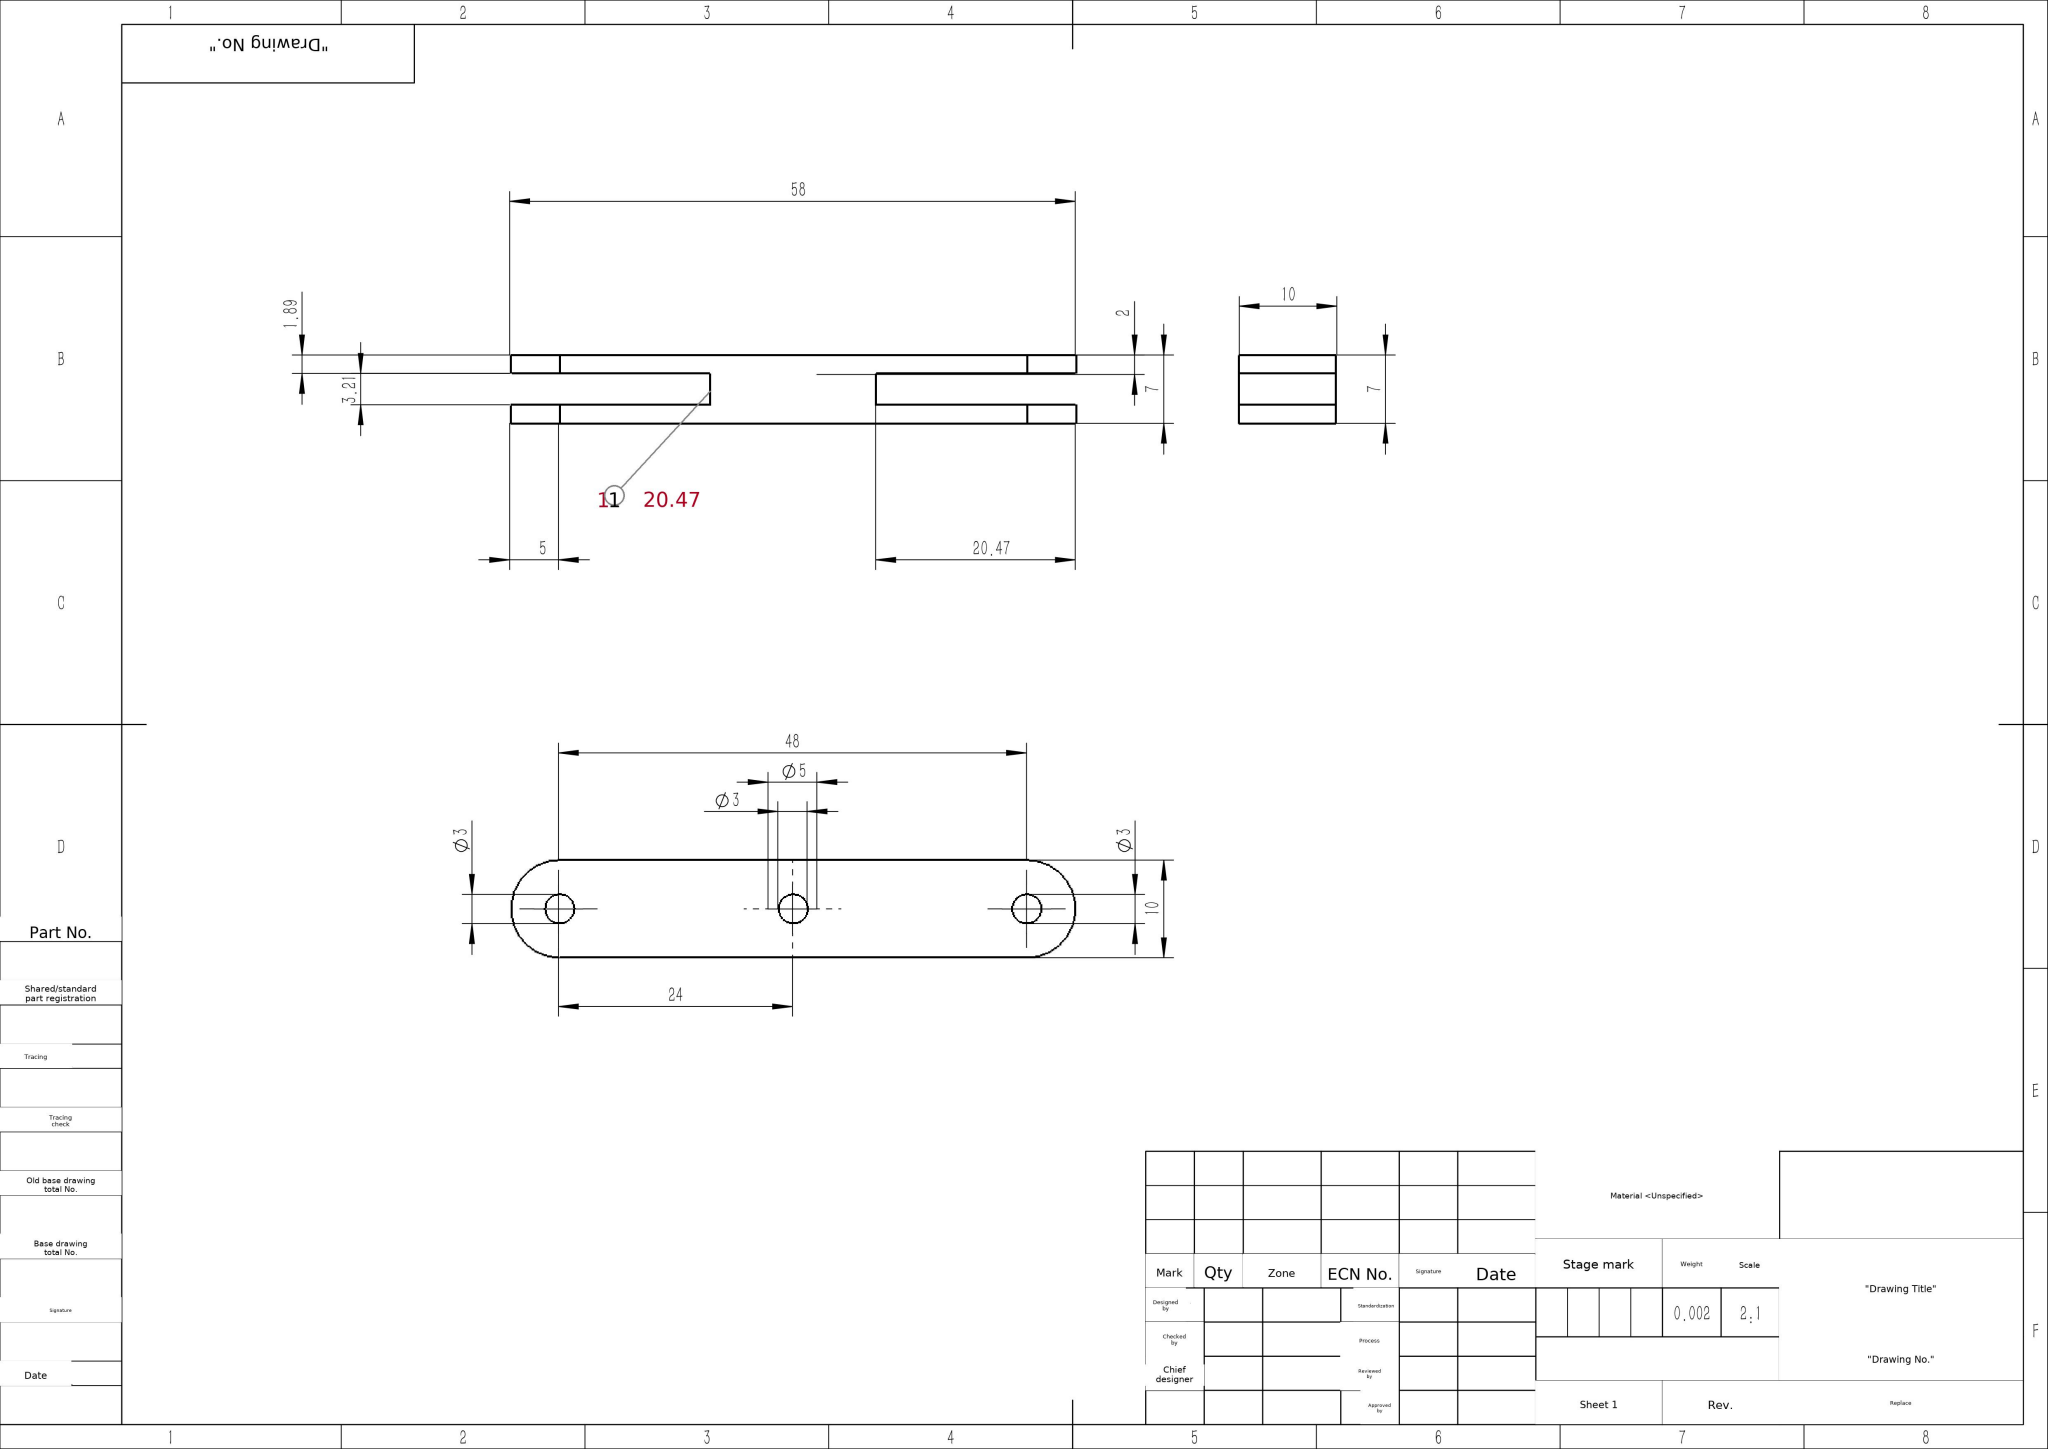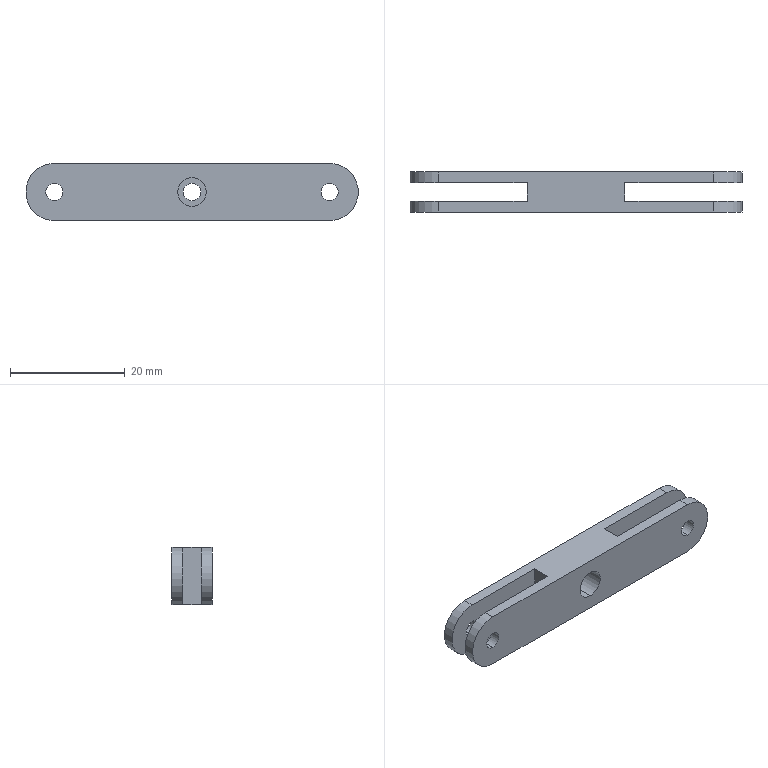Part | SolidWorks | mm | material <Unspecified> | 1 solid | 27 faces | box 58 x 7 x 10 mm | volume 2498 mm3 | cylinder 16 | plane 11 | commonest cylinder face diameters 3 x10 10 x4 5 x2
build123d program:
from build123d import *

# Parameters (mm, degrees)
SKETCH1_R           = 1.5
SKETCH1_R_2         = 2.5
BOSS_EXTRUDE1_DEPTH = 7
BOSS_EXTRUDE2_START = -2
SKETCH2_R           = 2.5
SKETCH2_R_2         = 1.5
BOSS_EXTRUDE2_DEPTH = 2
CUT_EXTRUDE1_DEPTH  = 10


with BuildPart() as part:
    # Sketch1 → Boss-Extrude1 (new body)
    with BuildSketch(Plane(origin=(0, 0, 0), x_dir=(1, 0, 0), z_dir=(0, 1, 0))):
        with BuildLine():
            Line((-24, 5), (24, 5))
            ThreePointArc((24, 5), (29, 0), (24, -5))
            Line((24, -5), (-24, -5))
            ThreePointArc((-24, -5), (-29, 0), (-24, 5))
        make_face()
        with Locations(Location((-24, 0, 0), (0, 0, 270))):
            Circle(SKETCH1_R, mode=Mode.SUBTRACT)
        with Locations(Location((24, 0, 0), (0, 0, 270))):
            Circle(SKETCH1_R, mode=Mode.SUBTRACT)
        with Locations(Location((0, 0, 0), (0, 0, 270))):
            Circle(SKETCH1_R_2, mode=Mode.SUBTRACT)
    extrude(amount=BOSS_EXTRUDE1_DEPTH)

    # Sketch2 → Boss-Extrude2 (add)
    with BuildSketch(Plane(origin=(0, 7, 0), x_dir=(1, 0, 0), z_dir=(0, 1, 0)).offset(BOSS_EXTRUDE2_START)):
        with Locations(Location((0, 0, 0), (0, 0, 270))):
            Circle(SKETCH2_R)
        with Locations(Location((0, 0, 0), (0, 0, 270))):
            Circle(SKETCH2_R_2, mode=Mode.SUBTRACT)
    extrude(amount=BOSS_EXTRUDE2_DEPTH)

    # Sketch3 → Cut-Extrude1 (cut)
    with BuildSketch(Plane(origin=(0, 0, -5), x_dir=(-1, 0, 0), z_dir=(0, 0, -1))):
        Polygon((-29, 5.106), (-11.241, 5.106), (-8.531, 5.106), (-8.531, 1.894), (-11.241, 1.894), (-29, 1.894), align=None)
        Polygon((29, 5.106), (11.241, 5.106), (8.531, 5.106), (8.531, 1.894), (11.241, 1.894), (29, 1.894), align=None)
    extrude(amount=-CUT_EXTRUDE1_DEPTH, mode=Mode.SUBTRACT)


solid = part.part
STEP:
#1=CARTESIAN_POINT('',(0.,5.,-1.5));
#2=VERTEX_POINT('',#1);
#3=CARTESIAN_POINT('',(0.,5.,1.5));
#4=VERTEX_POINT('',#3);
#5=CARTESIAN_POINT('',(0.,5.,0.));
#6=DIRECTION('',(0.,1.,0.));
#7=DIRECTION('',(0.,0.,1.));
#8=AXIS2_PLACEMENT_3D('',#5,#6,#7);
#9=CIRCLE('',#8,1.5);
#10=EDGE_CURVE('',#2,#4,#9,.T.);
#11=ORIENTED_EDGE('',*,*,#10,.F.);
#12=CARTESIAN_POINT('',(0.,7.,-1.5));
#13=VERTEX_POINT('',#12);
#14=CARTESIAN_POINT('',(0.,5.,-1.5));
#15=DIRECTION('',(0.,1.,0.));
#16=VECTOR('',#15,1000.);
#17=LINE('',#14,#16);
#18=EDGE_CURVE('',#2,#13,#17,.T.);
#19=ORIENTED_EDGE('',*,*,#18,.T.);
#20=CARTESIAN_POINT('',(0.,7.,1.5));
#21=VERTEX_POINT('',#20);
#22=CARTESIAN_POINT('',(0.,7.,0.));
#23=DIRECTION('',(0.,1.,0.));
#24=DIRECTION('',(0.,0.,1.));
#25=AXIS2_PLACEMENT_3D('',#22,#23,#24);
#26=CIRCLE('',#25,1.5);
#27=EDGE_CURVE('',#13,#21,#26,.T.);
#28=ORIENTED_EDGE('',*,*,#27,.T.);
#29=CARTESIAN_POINT('',(0.,5.,1.5));
#30=DIRECTION('',(0.,1.,0.));
#31=VECTOR('',#30,1000.);
#32=LINE('',#29,#31);
#33=EDGE_CURVE('',#4,#21,#32,.T.);
#34=ORIENTED_EDGE('',*,*,#33,.F.);
#35=EDGE_LOOP('',(#11,#19,#28,#34));
#36=FACE_OUTER_BOUND('',#35,.T.);
#37=CARTESIAN_POINT('',(0.,5.,0.));
#38=DIRECTION('',(0.,1.,0.));
#39=DIRECTION('',(0.,0.,1.));
#40=AXIS2_PLACEMENT_3D('',#37,#38,#39);
#41=CYLINDRICAL_SURFACE('',#40,1.5);
#42=ADVANCED_FACE('',(#36),#41,.F.);
#43=CARTESIAN_POINT('',(24.,1.894,1.5));
#44=VERTEX_POINT('',#43);
#45=CARTESIAN_POINT('',(24.,1.894,-1.5));
#46=VERTEX_POINT('',#45);
#47=CARTESIAN_POINT('',(24.,1.894,0.));
#48=DIRECTION('',(0.,-1.,0.));
#49=DIRECTION('',(0.,0.,-1.));
#50=AXIS2_PLACEMENT_3D('',#47,#48,#49);
#51=CIRCLE('',#50,1.5);
#52=EDGE_CURVE('',#44,#46,#51,.T.);
#53=ORIENTED_EDGE('',*,*,#52,.F.);
#54=CARTESIAN_POINT('',(24.,0.,1.5));
#55=VERTEX_POINT('',#54);
#56=CARTESIAN_POINT('',(24.,7.,1.5));
#57=DIRECTION('',(0.,-1.,0.));
#58=VECTOR('',#57,1000.);
#59=LINE('',#56,#58);
#60=EDGE_CURVE('',#44,#55,#59,.T.);
#61=ORIENTED_EDGE('',*,*,#60,.T.);
#62=CARTESIAN_POINT('',(24.,0.,-1.5));
#63=VERTEX_POINT('',#62);
#64=CARTESIAN_POINT('',(24.,0.,0.));
#65=DIRECTION('',(0.,1.,0.));
#66=DIRECTION('',(0.,0.,1.));
#67=AXIS2_PLACEMENT_3D('',#64,#65,#66);
#68=CIRCLE('',#67,1.5);
#69=EDGE_CURVE('',#63,#55,#68,.T.);
#70=ORIENTED_EDGE('',*,*,#69,.F.);
#71=CARTESIAN_POINT('',(24.,7.,-1.5));
#72=DIRECTION('',(0.,-1.,0.));
#73=VECTOR('',#72,1000.);
#74=LINE('',#71,#73);
#75=EDGE_CURVE('',#46,#63,#74,.T.);
#76=ORIENTED_EDGE('',*,*,#75,.F.);
#77=EDGE_LOOP('',(#53,#61,#70,#76));
#78=FACE_OUTER_BOUND('',#77,.T.);
#79=CARTESIAN_POINT('',(24.,7.,0.));
#80=DIRECTION('',(0.,-1.,0.));
#81=DIRECTION('',(0.,0.,-1.));
#82=AXIS2_PLACEMENT_3D('',#79,#80,#81);
#83=CYLINDRICAL_SURFACE('',#82,1.5);
#84=ADVANCED_FACE('',(#78),#83,.F.);
#85=CARTESIAN_POINT('',(-24.,7.,-1.5));
#86=VERTEX_POINT('',#85);
#87=CARTESIAN_POINT('',(-24.,7.,1.5));
#88=VERTEX_POINT('',#87);
#89=CARTESIAN_POINT('',(-24.,7.,0.));
#90=DIRECTION('',(0.,1.,0.));
#91=DIRECTION('',(0.,0.,1.));
#92=AXIS2_PLACEMENT_3D('',#89,#90,#91);
#93=CIRCLE('',#92,1.5);
#94=EDGE_CURVE('',#86,#88,#93,.T.);
#95=ORIENTED_EDGE('',*,*,#94,.T.);
#96=CARTESIAN_POINT('',(-24.,5.106,1.5));
#97=VERTEX_POINT('',#96);
#98=CARTESIAN_POINT('',(-24.,7.,1.5));
#99=DIRECTION('',(0.,-1.,0.));
#100=VECTOR('',#99,1000.);
#101=LINE('',#98,#100);
#102=EDGE_CURVE('',#88,#97,#101,.T.);
#103=ORIENTED_EDGE('',*,*,#102,.T.);
#104=CARTESIAN_POINT('',(-24.,5.106,-1.5));
#105=VERTEX_POINT('',#104);
#106=CARTESIAN_POINT('',(-24.,5.106,0.));
#107=DIRECTION('',(0.,1.,0.));
#108=DIRECTION('',(0.,0.,1.));
#109=AXIS2_PLACEMENT_3D('',#106,#107,#108);
#110=CIRCLE('',#109,1.5);
#111=EDGE_CURVE('',#105,#97,#110,.T.);
#112=ORIENTED_EDGE('',*,*,#111,.F.);
#113=CARTESIAN_POINT('',(-24.,7.,-1.5));
#114=DIRECTION('',(0.,-1.,0.));
#115=VECTOR('',#114,1000.);
#116=LINE('',#113,#115);
#117=EDGE_CURVE('',#86,#105,#116,.T.);
#118=ORIENTED_EDGE('',*,*,#117,.F.);
#119=EDGE_LOOP('',(#95,#103,#112,#118));
#120=FACE_OUTER_BOUND('',#119,.T.);
#121=CARTESIAN_POINT('',(-24.,7.,0.));
#122=DIRECTION('',(0.,-1.,0.));
#123=DIRECTION('',(0.,0.,-1.));
#124=AXIS2_PLACEMENT_3D('',#121,#122,#123);
#125=CYLINDRICAL_SURFACE('',#124,1.5);
#126=ADVANCED_FACE('',(#120),#125,.F.);
#127=CARTESIAN_POINT('',(0.,5.,-2.5));
#128=VERTEX_POINT('',#127);
#129=CARTESIAN_POINT('',(0.,5.,2.5));
#130=VERTEX_POINT('',#129);
#131=CARTESIAN_POINT('',(0.,5.,0.));
#132=DIRECTION('',(0.,1.,0.));
#133=DIRECTION('',(0.,0.,1.));
#134=AXIS2_PLACEMENT_3D('',#131,#132,#133);
#135=CIRCLE('',#134,2.5);
#136=EDGE_CURVE('',#128,#130,#135,.T.);
#137=ORIENTED_EDGE('',*,*,#136,.T.);
#138=CARTESIAN_POINT('',(0.,0.,2.5));
#139=VERTEX_POINT('',#138);
#140=CARTESIAN_POINT('',(0.,7.,2.5));
#141=DIRECTION('',(0.,-1.,0.));
#142=VECTOR('',#141,1000.);
#143=LINE('',#140,#142);
#144=EDGE_CURVE('',#130,#139,#143,.T.);
#145=ORIENTED_EDGE('',*,*,#144,.T.);
#146=CARTESIAN_POINT('',(0.,0.,-2.5));
#147=VERTEX_POINT('',#146);
#148=CARTESIAN_POINT('',(0.,0.,0.));
#149=DIRECTION('',(0.,1.,0.));
#150=DIRECTION('',(0.,0.,1.));
#151=AXIS2_PLACEMENT_3D('',#148,#149,#150);
#152=CIRCLE('',#151,2.5);
#153=EDGE_CURVE('',#147,#139,#152,.T.);
#154=ORIENTED_EDGE('',*,*,#153,.F.);
#155=CARTESIAN_POINT('',(0.,7.,-2.5));
#156=DIRECTION('',(0.,-1.,0.));
#157=VECTOR('',#156,1000.);
#158=LINE('',#155,#157);
#159=EDGE_CURVE('',#128,#147,#158,.T.);
#160=ORIENTED_EDGE('',*,*,#159,.F.);
#161=EDGE_LOOP('',(#137,#145,#154,#160));
#162=FACE_OUTER_BOUND('',#161,.T.);
#163=CARTESIAN_POINT('',(0.,7.,0.));
#164=DIRECTION('',(0.,-1.,0.));
#165=DIRECTION('',(0.,0.,-1.));
#166=AXIS2_PLACEMENT_3D('',#163,#164,#165);
#167=CYLINDRICAL_SURFACE('',#166,2.5);
#168=ADVANCED_FACE('',(#162),#167,.F.);
#169=CARTESIAN_POINT('',(24.,7.,-1.5));
#170=VERTEX_POINT('',#169);
#171=CARTESIAN_POINT('',(24.,7.,1.5));
#172=VERTEX_POINT('',#171);
#173=CARTESIAN_POINT('',(24.,7.,0.));
#174=DIRECTION('',(0.,1.,0.));
#175=DIRECTION('',(0.,0.,1.));
#176=AXIS2_PLACEMENT_3D('',#173,#174,#175);
#177=CIRCLE('',#176,1.5);
#178=EDGE_CURVE('',#170,#172,#177,.T.);
#179=ORIENTED_EDGE('',*,*,#178,.T.);
#180=CARTESIAN_POINT('',(24.,5.106,1.5));
#181=VERTEX_POINT('',#180);
#182=CARTESIAN_POINT('',(24.,7.,1.5));
#183=DIRECTION('',(0.,-1.,0.));
#184=VECTOR('',#183,1000.);
#185=LINE('',#182,#184);
#186=EDGE_CURVE('',#172,#181,#185,.T.);
#187=ORIENTED_EDGE('',*,*,#186,.T.);
#188=CARTESIAN_POINT('',(24.,5.106,-1.5));
#189=VERTEX_POINT('',#188);
#190=CARTESIAN_POINT('',(24.,5.106,0.));
#191=DIRECTION('',(0.,1.,0.));
#192=DIRECTION('',(0.,0.,1.));
#193=AXIS2_PLACEMENT_3D('',#190,#191,#192);
#194=CIRCLE('',#193,1.5);
#195=EDGE_CURVE('',#189,#181,#194,.T.);
#196=ORIENTED_EDGE('',*,*,#195,.F.);
#197=CARTESIAN_POINT('',(24.,7.,-1.5));
#198=DIRECTION('',(0.,-1.,0.));
#199=VECTOR('',#198,1000.);
#200=LINE('',#197,#199);
#201=EDGE_CURVE('',#170,#189,#200,.T.);
#202=ORIENTED_EDGE('',*,*,#201,.F.);
#203=EDGE_LOOP('',(#179,#187,#196,#202));
#204=FACE_OUTER_BOUND('',#203,.T.);
#205=CARTESIAN_POINT('',(24.,7.,0.));
#206=DIRECTION('',(0.,-1.,0.));
#207=DIRECTION('',(0.,0.,-1.));
#208=AXIS2_PLACEMENT_3D('',#205,#206,#207);
#209=CYLINDRICAL_SURFACE('',#208,1.5);
#210=ADVANCED_FACE('',(#204),#209,.F.);
#211=CARTESIAN_POINT('',(-24.,1.894,1.5));
#212=VERTEX_POINT('',#211);
#213=CARTESIAN_POINT('',(-24.,1.894,-1.5));
#214=VERTEX_POINT('',#213);
#215=CARTESIAN_POINT('',(-24.,1.894,0.));
#216=DIRECTION('',(0.,-1.,0.));
#217=DIRECTION('',(0.,0.,-1.));
#218=AXIS2_PLACEMENT_3D('',#215,#216,#217);
#219=CIRCLE('',#218,1.5);
#220=EDGE_CURVE('',#212,#214,#219,.T.);
#221=ORIENTED_EDGE('',*,*,#220,.F.);
#222=CARTESIAN_POINT('',(-24.,0.,1.5));
#223=VERTEX_POINT('',#222);
#224=CARTESIAN_POINT('',(-24.,7.,1.5));
#225=DIRECTION('',(0.,-1.,0.));
#226=VECTOR('',#225,1000.);
#227=LINE('',#224,#226);
#228=EDGE_CURVE('',#212,#223,#227,.T.);
#229=ORIENTED_EDGE('',*,*,#228,.T.);
#230=CARTESIAN_POINT('',(-24.,0.,-1.5));
#231=VERTEX_POINT('',#230);
#232=CARTESIAN_POINT('',(-24.,0.,0.));
#233=DIRECTION('',(0.,1.,0.));
#234=DIRECTION('',(0.,0.,1.));
#235=AXIS2_PLACEMENT_3D('',#232,#233,#234);
#236=CIRCLE('',#235,1.5);
#237=EDGE_CURVE('',#231,#223,#236,.T.);
#238=ORIENTED_EDGE('',*,*,#237,.F.);
#239=CARTESIAN_POINT('',(-24.,7.,-1.5));
#240=DIRECTION('',(0.,-1.,0.));
#241=VECTOR('',#240,1000.);
#242=LINE('',#239,#241);
#243=EDGE_CURVE('',#214,#231,#242,.T.);
#244=ORIENTED_EDGE('',*,*,#243,.F.);
#245=EDGE_LOOP('',(#221,#229,#238,#244));
#246=FACE_OUTER_BOUND('',#245,.T.);
#247=CARTESIAN_POINT('',(-24.,7.,0.));
#248=DIRECTION('',(0.,-1.,0.));
#249=DIRECTION('',(0.,0.,-1.));
#250=AXIS2_PLACEMENT_3D('',#247,#248,#249);
#251=CYLINDRICAL_SURFACE('',#250,1.5);
#252=ADVANCED_FACE('',(#246),#251,.F.);
#253=CARTESIAN_POINT('',(-24.,1.894,5.));
#254=VERTEX_POINT('',#253);
#255=CARTESIAN_POINT('',(-24.,0.,5.));
#256=VERTEX_POINT('',#255);
#257=CARTESIAN_POINT('',(-24.,7.,5.));
#258=DIRECTION('',(0.,-1.,0.));
#259=VECTOR('',#258,1000.);
#260=LINE('',#257,#259);
#261=EDGE_CURVE('',#254,#256,#260,.T.);
#262=ORIENTED_EDGE('',*,*,#261,.F.);
#263=CARTESIAN_POINT('',(-24.,1.894,-5.));
#264=VERTEX_POINT('',#263);
#265=CARTESIAN_POINT('',(-24.,1.894,0.));
#266=DIRECTION('',(0.,-1.,0.));
#267=DIRECTION('',(0.,0.,-1.));
#268=AXIS2_PLACEMENT_3D('',#265,#266,#267);
#269=CIRCLE('',#268,5.);
#270=EDGE_CURVE('',#254,#264,#269,.T.);
#271=ORIENTED_EDGE('',*,*,#270,.T.);
#272=CARTESIAN_POINT('',(-24.,0.,-5.));
#273=VERTEX_POINT('',#272);
#274=CARTESIAN_POINT('',(-24.,7.,-5.));
#275=DIRECTION('',(0.,-1.,0.));
#276=VECTOR('',#275,1000.);
#277=LINE('',#274,#276);
#278=EDGE_CURVE('',#264,#273,#277,.T.);
#279=ORIENTED_EDGE('',*,*,#278,.T.);
#280=CARTESIAN_POINT('',(-24.,0.,0.));
#281=DIRECTION('',(0.,1.,0.));
#282=DIRECTION('',(0.,0.,1.));
#283=AXIS2_PLACEMENT_3D('',#280,#281,#282);
#284=CIRCLE('',#283,5.);
#285=EDGE_CURVE('',#273,#256,#284,.T.);
#286=ORIENTED_EDGE('',*,*,#285,.T.);
#287=EDGE_LOOP('',(#262,#271,#279,#286));
#288=FACE_OUTER_BOUND('',#287,.T.);
#289=CARTESIAN_POINT('',(-24.,7.,0.));
#290=DIRECTION('',(0.,-1.,0.));
#291=DIRECTION('',(0.,0.,-1.));
#292=AXIS2_PLACEMENT_3D('',#289,#290,#291);
#293=CYLINDRICAL_SURFACE('',#292,5.);
#294=ADVANCED_FACE('',(#288),#293,.T.);
#295=CARTESIAN_POINT('',(24.,7.,5.));
#296=VERTEX_POINT('',#295);
#297=CARTESIAN_POINT('',(24.,5.106,5.));
#298=VERTEX_POINT('',#297);
#299=CARTESIAN_POINT('',(24.,7.,5.));
#300=DIRECTION('',(0.,-1.,0.));
#301=VECTOR('',#300,1000.);
#302=LINE('',#299,#301);
#303=EDGE_CURVE('',#296,#298,#302,.T.);
#304=ORIENTED_EDGE('',*,*,#303,.T.);
#305=CARTESIAN_POINT('',(24.,5.106,-5.));
#306=VERTEX_POINT('',#305);
#307=CARTESIAN_POINT('',(24.,5.106,0.));
#308=DIRECTION('',(0.,1.,0.));
#309=DIRECTION('',(0.,0.,1.));
#310=AXIS2_PLACEMENT_3D('',#307,#308,#309);
#311=CIRCLE('',#310,5.);
#312=EDGE_CURVE('',#298,#306,#311,.T.);
#313=ORIENTED_EDGE('',*,*,#312,.T.);
#314=CARTESIAN_POINT('',(24.,7.,-5.));
#315=VERTEX_POINT('',#314);
#316=CARTESIAN_POINT('',(24.,7.,-5.));
#317=DIRECTION('',(0.,-1.,0.));
#318=VECTOR('',#317,1000.);
#319=LINE('',#316,#318);
#320=EDGE_CURVE('',#315,#306,#319,.T.);
#321=ORIENTED_EDGE('',*,*,#320,.F.);
#322=CARTESIAN_POINT('',(24.,7.,0.));
#323=DIRECTION('',(0.,1.,0.));
#324=DIRECTION('',(0.,0.,-1.));
#325=AXIS2_PLACEMENT_3D('',#322,#323,#324);
#326=CIRCLE('',#325,5.);
#327=EDGE_CURVE('',#296,#315,#326,.T.);
#328=ORIENTED_EDGE('',*,*,#327,.F.);
#329=EDGE_LOOP('',(#304,#313,#321,#328));
#330=FACE_OUTER_BOUND('',#329,.T.);
#331=CARTESIAN_POINT('',(24.,7.,0.));
#332=DIRECTION('',(0.,-1.,0.));
#333=DIRECTION('',(0.,0.,-1.));
#334=AXIS2_PLACEMENT_3D('',#331,#332,#333);
#335=CYLINDRICAL_SURFACE('',#334,5.);
#336=ADVANCED_FACE('',(#330),#335,.T.);
#337=ORIENTED_EDGE('',*,*,#228,.F.);
#338=CARTESIAN_POINT('',(-24.,1.894,0.));
#339=DIRECTION('',(0.,-1.,0.));
#340=DIRECTION('',(0.,0.,-1.));
#341=AXIS2_PLACEMENT_3D('',#338,#339,#340);
#342=CIRCLE('',#341,1.5);
#343=EDGE_CURVE('',#214,#212,#342,.T.);
#344=ORIENTED_EDGE('',*,*,#343,.F.);
#345=ORIENTED_EDGE('',*,*,#243,.T.);
#346=CARTESIAN_POINT('',(-24.,0.,0.));
#347=DIRECTION('',(0.,1.,0.));
#348=DIRECTION('',(0.,0.,1.));
#349=AXIS2_PLACEMENT_3D('',#346,#347,#348);
#350=CIRCLE('',#349,1.5);
#351=EDGE_CURVE('',#223,#231,#350,.T.);
#352=ORIENTED_EDGE('',*,*,#351,.F.);
#353=EDGE_LOOP('',(#337,#344,#345,#352));
#354=FACE_OUTER_BOUND('',#353,.T.);
#355=CARTESIAN_POINT('',(-24.,7.,0.));
#356=DIRECTION('',(0.,-1.,0.));
#357=DIRECTION('',(0.,0.,-1.));
#358=AXIS2_PLACEMENT_3D('',#355,#356,#357);
#359=CYLINDRICAL_SURFACE('',#358,1.5);
#360=ADVANCED_FACE('',(#354),#359,.F.);
#361=ORIENTED_EDGE('',*,*,#186,.F.);
#362=CARTESIAN_POINT('',(24.,7.,0.));
#363=DIRECTION('',(0.,1.,0.));
#364=DIRECTION('',(0.,0.,1.));
#365=AXIS2_PLACEMENT_3D('',#362,#363,#364);
#366=CIRCLE('',#365,1.5);
#367=EDGE_CURVE('',#172,#170,#366,.T.);
#368=ORIENTED_EDGE('',*,*,#367,.T.);
#369=ORIENTED_EDGE('',*,*,#201,.T.);
#370=CARTESIAN_POINT('',(24.,5.106,0.));
#371=DIRECTION('',(0.,1.,0.));
#372=DIRECTION('',(0.,0.,1.));
#373=AXIS2_PLACEMENT_3D('',#370,#371,#372);
#374=CIRCLE('',#373,1.5);
#375=EDGE_CURVE('',#181,#189,#374,.T.);
#376=ORIENTED_EDGE('',*,*,#375,.F.);
#377=EDGE_LOOP('',(#361,#368,#369,#376));
#378=FACE_OUTER_BOUND('',#377,.T.);
#379=CARTESIAN_POINT('',(24.,7.,0.));
#380=DIRECTION('',(0.,-1.,0.));
#381=DIRECTION('',(0.,0.,-1.));
#382=AXIS2_PLACEMENT_3D('',#379,#380,#381);
#383=CYLINDRICAL_SURFACE('',#382,1.5);
#384=ADVANCED_FACE('',(#378),#383,.F.);
#385=ORIENTED_EDGE('',*,*,#144,.F.);
#386=CARTESIAN_POINT('',(0.,5.,0.));
#387=DIRECTION('',(0.,1.,0.));
#388=DIRECTION('',(0.,0.,1.));
#389=AXIS2_PLACEMENT_3D('',#386,#387,#388);
#390=CIRCLE('',#389,2.5);
#391=EDGE_CURVE('',#130,#128,#390,.T.);
#392=ORIENTED_EDGE('',*,*,#391,.T.);
#393=ORIENTED_EDGE('',*,*,#159,.T.);
#394=CARTESIAN_POINT('',(0.,0.,0.));
#395=DIRECTION('',(0.,1.,0.));
#396=DIRECTION('',(0.,0.,1.));
#397=AXIS2_PLACEMENT_3D('',#394,#395,#396);
#398=CIRCLE('',#397,2.5);
#399=EDGE_CURVE('',#139,#147,#398,.T.);
#400=ORIENTED_EDGE('',*,*,#399,.F.);
#401=EDGE_LOOP('',(#385,#392,#393,#400));
#402=FACE_OUTER_BOUND('',#401,.T.);
#403=CARTESIAN_POINT('',(0.,7.,0.));
#404=DIRECTION('',(0.,-1.,0.));
#405=DIRECTION('',(0.,0.,-1.));
#406=AXIS2_PLACEMENT_3D('',#403,#404,#405);
#407=CYLINDRICAL_SURFACE('',#406,2.5);
#408=ADVANCED_FACE('',(#402),#407,.F.);
#409=ORIENTED_EDGE('',*,*,#178,.F.);
#410=ORIENTED_EDGE('',*,*,#367,.F.);
#411=EDGE_LOOP('',(#409,#410));
#412=FACE_BOUND('',#411,.T.);
#413=CARTESIAN_POINT('',(-24.,7.,-5.));
#414=VERTEX_POINT('',#413);
#415=CARTESIAN_POINT('',(-24.,7.,5.));
#416=VERTEX_POINT('',#415);
#417=CARTESIAN_POINT('',(-24.,7.,0.));
#418=DIRECTION('',(0.,1.,0.));
#419=DIRECTION('',(0.,0.,1.));
#420=AXIS2_PLACEMENT_3D('',#417,#418,#419);
#421=CIRCLE('',#420,5.);
#422=EDGE_CURVE('',#414,#416,#421,.T.);
#423=ORIENTED_EDGE('',*,*,#422,.T.);
#424=CARTESIAN_POINT('',(-24.,7.,5.));
#425=DIRECTION('',(1.,0.,0.));
#426=VECTOR('',#425,1000.);
#427=LINE('',#424,#426);
#428=EDGE_CURVE('',#416,#296,#427,.T.);
#429=ORIENTED_EDGE('',*,*,#428,.T.);
#430=ORIENTED_EDGE('',*,*,#327,.T.);
#431=CARTESIAN_POINT('',(-24.,7.,-5.));
#432=DIRECTION('',(-1.,0.,0.));
#433=VECTOR('',#432,1000.);
#434=LINE('',#431,#433);
#435=EDGE_CURVE('',#315,#414,#434,.T.);
#436=ORIENTED_EDGE('',*,*,#435,.T.);
#437=EDGE_LOOP('',(#423,#429,#430,#436));
#438=FACE_OUTER_BOUND('',#437,.T.);
#439=ORIENTED_EDGE('',*,*,#94,.F.);
#440=CARTESIAN_POINT('',(-24.,7.,0.));
#441=DIRECTION('',(0.,1.,0.));
#442=DIRECTION('',(0.,0.,1.));
#443=AXIS2_PLACEMENT_3D('',#440,#441,#442);
#444=CIRCLE('',#443,1.5);
#445=EDGE_CURVE('',#88,#86,#444,.T.);
#446=ORIENTED_EDGE('',*,*,#445,.F.);
#447=EDGE_LOOP('',(#439,#446));
#448=FACE_BOUND('',#447,.T.);
#449=CARTESIAN_POINT('',(0.,7.,0.));
#450=DIRECTION('',(0.,1.,0.));
#451=DIRECTION('',(0.,0.,1.));
#452=AXIS2_PLACEMENT_3D('',#449,#450,#451);
#453=CIRCLE('',#452,1.5);
#454=EDGE_CURVE('',#21,#13,#453,.T.);
#455=ORIENTED_EDGE('',*,*,#454,.F.);
#456=ORIENTED_EDGE('',*,*,#27,.F.);
#457=EDGE_LOOP('',(#455,#456));
#458=FACE_BOUND('',#457,.T.);
#459=CARTESIAN_POINT('',(-24.,7.,0.));
#460=DIRECTION('',(0.,1.,0.));
#461=DIRECTION('',(0.,0.,1.));
#462=AXIS2_PLACEMENT_3D('',#459,#460,#461);
#463=PLANE('',#462);
#464=ADVANCED_FACE('',(#412,#438,#448,#458),#463,.T.);
#465=ORIENTED_EDGE('',*,*,#285,.F.);
#466=CARTESIAN_POINT('',(24.,0.,-5.));
#467=VERTEX_POINT('',#466);
#468=CARTESIAN_POINT('',(-24.,0.,-5.));
#469=DIRECTION('',(-1.,0.,0.));
#470=VECTOR('',#469,1000.);
#471=LINE('',#468,#470);
#472=EDGE_CURVE('',#467,#273,#471,.T.);
#473=ORIENTED_EDGE('',*,*,#472,.F.);
#474=CARTESIAN_POINT('',(24.,0.,5.));
#475=VERTEX_POINT('',#474);
#476=CARTESIAN_POINT('',(24.,0.,0.));
#477=DIRECTION('',(0.,1.,0.));
#478=DIRECTION('',(0.,0.,-1.));
#479=AXIS2_PLACEMENT_3D('',#476,#477,#478);
#480=CIRCLE('',#479,5.);
#481=EDGE_CURVE('',#475,#467,#480,.T.);
#482=ORIENTED_EDGE('',*,*,#481,.F.);
#483=CARTESIAN_POINT('',(-24.,0.,5.));
#484=DIRECTION('',(1.,0.,0.));
#485=VECTOR('',#484,1000.);
#486=LINE('',#483,#485);
#487=EDGE_CURVE('',#256,#475,#486,.T.);
#488=ORIENTED_EDGE('',*,*,#487,.F.);
#489=EDGE_LOOP('',(#465,#473,#482,#488));
#490=FACE_OUTER_BOUND('',#489,.T.);
#491=ORIENTED_EDGE('',*,*,#237,.T.);
#492=ORIENTED_EDGE('',*,*,#351,.T.);
#493=EDGE_LOOP('',(#491,#492));
#494=FACE_BOUND('',#493,.T.);
#495=ORIENTED_EDGE('',*,*,#69,.T.);
#496=CARTESIAN_POINT('',(24.,0.,0.));
#497=DIRECTION('',(0.,1.,0.));
#498=DIRECTION('',(0.,0.,1.));
#499=AXIS2_PLACEMENT_3D('',#496,#497,#498);
#500=CIRCLE('',#499,1.5);
#501=EDGE_CURVE('',#55,#63,#500,.T.);
#502=ORIENTED_EDGE('',*,*,#501,.T.);
#503=EDGE_LOOP('',(#495,#502));
#504=FACE_BOUND('',#503,.T.);
#505=ORIENTED_EDGE('',*,*,#153,.T.);
#506=ORIENTED_EDGE('',*,*,#399,.T.);
#507=EDGE_LOOP('',(#505,#506));
#508=FACE_BOUND('',#507,.T.);
#509=CARTESIAN_POINT('',(-24.,0.,0.));
#510=DIRECTION('',(0.,1.,0.));
#511=DIRECTION('',(0.,0.,1.));
#512=AXIS2_PLACEMENT_3D('',#509,#510,#511);
#513=PLANE('',#512);
#514=ADVANCED_FACE('',(#490,#494,#504,#508),#513,.F.);
#515=CARTESIAN_POINT('',(-24.,5.106,-5.));
#516=VERTEX_POINT('',#515);
#517=CARTESIAN_POINT('',(-24.,7.,-5.));
#518=DIRECTION('',(0.,-1.,0.));
#519=VECTOR('',#518,1000.);
#520=LINE('',#517,#519);
#521=EDGE_CURVE('',#414,#516,#520,.T.);
#522=ORIENTED_EDGE('',*,*,#521,.T.);
#523=CARTESIAN_POINT('',(-24.,5.106,5.));
#524=VERTEX_POINT('',#523);
#525=CARTESIAN_POINT('',(-24.,5.106,0.));
#526=DIRECTION('',(0.,1.,0.));
#527=DIRECTION('',(0.,0.,1.));
#528=AXIS2_PLACEMENT_3D('',#525,#526,#527);
#529=CIRCLE('',#528,5.);
#530=EDGE_CURVE('',#516,#524,#529,.T.);
#531=ORIENTED_EDGE('',*,*,#530,.T.);
#532=CARTESIAN_POINT('',(-24.,7.,5.));
#533=DIRECTION('',(0.,-1.,0.));
#534=VECTOR('',#533,1000.);
#535=LINE('',#532,#534);
#536=EDGE_CURVE('',#416,#524,#535,.T.);
#537=ORIENTED_EDGE('',*,*,#536,.F.);
#538=ORIENTED_EDGE('',*,*,#422,.F.);
#539=EDGE_LOOP('',(#522,#531,#537,#538));
#540=FACE_OUTER_BOUND('',#539,.T.);
#541=CARTESIAN_POINT('',(-24.,7.,0.));
#542=DIRECTION('',(0.,-1.,0.));
#543=DIRECTION('',(0.,0.,-1.));
#544=AXIS2_PLACEMENT_3D('',#541,#542,#543);
#545=CYLINDRICAL_SURFACE('',#544,5.);
#546=ADVANCED_FACE('',(#540),#545,.T.);
#547=CARTESIAN_POINT('',(8.531,5.106,5.));
#548=VERTEX_POINT('',#547);
#549=CARTESIAN_POINT('',(8.531,1.894,5.));
#550=VERTEX_POINT('',#549);
#551=CARTESIAN_POINT('',(8.531,5.106,5.));
#552=DIRECTION('',(0.,-1.,0.));
#553=VECTOR('',#552,1000.);
#554=LINE('',#551,#553);
#555=EDGE_CURVE('',#548,#550,#554,.T.);
#556=ORIENTED_EDGE('',*,*,#555,.F.);
#557=CARTESIAN_POINT('',(29.,5.106,5.));
#558=DIRECTION('',(-1.,0.,0.));
#559=VECTOR('',#558,1000.);
#560=LINE('',#557,#559);
#561=EDGE_CURVE('',#298,#548,#560,.T.);
#562=ORIENTED_EDGE('',*,*,#561,.F.);
#563=ORIENTED_EDGE('',*,*,#303,.F.);
#564=ORIENTED_EDGE('',*,*,#428,.F.);
#565=ORIENTED_EDGE('',*,*,#536,.T.);
#566=CARTESIAN_POINT('',(-8.531,5.106,5.));
#567=VERTEX_POINT('',#566);
#568=CARTESIAN_POINT('',(-11.241,5.106,5.));
#569=DIRECTION('',(-1.,0.,0.));
#570=VECTOR('',#569,1000.);
#571=LINE('',#568,#570);
#572=EDGE_CURVE('',#567,#524,#571,.T.);
#573=ORIENTED_EDGE('',*,*,#572,.F.);
#574=CARTESIAN_POINT('',(-8.531,1.894,5.));
#575=VERTEX_POINT('',#574);
#576=CARTESIAN_POINT('',(-8.531,5.106,5.));
#577=DIRECTION('',(0.,1.,0.));
#578=VECTOR('',#577,1000.);
#579=LINE('',#576,#578);
#580=EDGE_CURVE('',#575,#567,#579,.T.);
#581=ORIENTED_EDGE('',*,*,#580,.F.);
#582=CARTESIAN_POINT('',(-29.,1.894,5.));
#583=DIRECTION('',(1.,0.,0.));
#584=VECTOR('',#583,1000.);
#585=LINE('',#582,#584);
#586=EDGE_CURVE('',#254,#575,#585,.T.);
#587=ORIENTED_EDGE('',*,*,#586,.F.);
#588=ORIENTED_EDGE('',*,*,#261,.T.);
#589=ORIENTED_EDGE('',*,*,#487,.T.);
#590=CARTESIAN_POINT('',(24.,1.894,5.));
#591=VERTEX_POINT('',#590);
#592=CARTESIAN_POINT('',(24.,7.,5.));
#593=DIRECTION('',(0.,-1.,0.));
#594=VECTOR('',#593,1000.);
#595=LINE('',#592,#594);
#596=EDGE_CURVE('',#591,#475,#595,.T.);
#597=ORIENTED_EDGE('',*,*,#596,.F.);
#598=CARTESIAN_POINT('',(11.241,1.894,5.));
#599=DIRECTION('',(1.,0.,0.));
#600=VECTOR('',#599,1000.);
#601=LINE('',#598,#600);
#602=EDGE_CURVE('',#550,#591,#601,.T.);
#603=ORIENTED_EDGE('',*,*,#602,.F.);
#604=EDGE_LOOP('',(#556,#562,#563,#564,#565,#573,#581,#587,#588,#589,#597,#603));
#605=FACE_OUTER_BOUND('',#604,.T.);
#606=CARTESIAN_POINT('',(-24.,7.,5.));
#607=DIRECTION('',(0.,0.,-1.));
#608=DIRECTION('',(-1.,0.,0.));
#609=AXIS2_PLACEMENT_3D('',#606,#607,#608);
#610=PLANE('',#609);
#611=ADVANCED_FACE('',(#605),#610,.F.);
#612=CARTESIAN_POINT('',(24.,1.894,-5.));
#613=VERTEX_POINT('',#612);
#614=CARTESIAN_POINT('',(24.,7.,-5.));
#615=DIRECTION('',(0.,-1.,0.));
#616=VECTOR('',#615,1000.);
#617=LINE('',#614,#616);
#618=EDGE_CURVE('',#613,#467,#617,.T.);
#619=ORIENTED_EDGE('',*,*,#618,.F.);
#620=CARTESIAN_POINT('',(24.,1.894,0.));
#621=DIRECTION('',(0.,-1.,0.));
#622=DIRECTION('',(0.,0.,-1.));
#623=AXIS2_PLACEMENT_3D('',#620,#621,#622);
#624=CIRCLE('',#623,5.);
#625=EDGE_CURVE('',#613,#591,#624,.T.);
#626=ORIENTED_EDGE('',*,*,#625,.T.);
#627=ORIENTED_EDGE('',*,*,#596,.T.);
#628=ORIENTED_EDGE('',*,*,#481,.T.);
#629=EDGE_LOOP('',(#619,#626,#627,#628));
#630=FACE_OUTER_BOUND('',#629,.T.);
#631=CARTESIAN_POINT('',(24.,7.,0.));
#632=DIRECTION('',(0.,-1.,0.));
#633=DIRECTION('',(0.,0.,-1.));
#634=AXIS2_PLACEMENT_3D('',#631,#632,#633);
#635=CYLINDRICAL_SURFACE('',#634,5.);
#636=ADVANCED_FACE('',(#630),#635,.T.);
#637=ORIENTED_EDGE('',*,*,#320,.T.);
#638=CARTESIAN_POINT('',(8.531,5.106,-5.));
#639=VERTEX_POINT('',#638);
#640=CARTESIAN_POINT('',(29.,5.106,-5.));
#641=DIRECTION('',(1.,0.,0.));
#642=VECTOR('',#641,1000.);
#643=LINE('',#640,#642);
#644=EDGE_CURVE('',#639,#306,#643,.T.);
#645=ORIENTED_EDGE('',*,*,#644,.F.);
#646=CARTESIAN_POINT('',(8.531,1.894,-5.));
#647=VERTEX_POINT('',#646);
#648=CARTESIAN_POINT('',(8.531,5.106,-5.));
#649=DIRECTION('',(0.,1.,0.));
#650=VECTOR('',#649,1000.);
#651=LINE('',#648,#650);
#652=EDGE_CURVE('',#647,#639,#651,.T.);
#653=ORIENTED_EDGE('',*,*,#652,.F.);
#654=CARTESIAN_POINT('',(11.241,1.894,-5.));
#655=DIRECTION('',(-1.,0.,0.));
#656=VECTOR('',#655,1000.);
#657=LINE('',#654,#656);
#658=EDGE_CURVE('',#613,#647,#657,.T.);
#659=ORIENTED_EDGE('',*,*,#658,.F.);
#660=ORIENTED_EDGE('',*,*,#618,.T.);
#661=ORIENTED_EDGE('',*,*,#472,.T.);
#662=ORIENTED_EDGE('',*,*,#278,.F.);
#663=CARTESIAN_POINT('',(-8.531,1.894,-5.));
#664=VERTEX_POINT('',#663);
#665=CARTESIAN_POINT('',(-29.,1.894,-5.));
#666=DIRECTION('',(-1.,0.,0.));
#667=VECTOR('',#666,1000.);
#668=LINE('',#665,#667);
#669=EDGE_CURVE('',#664,#264,#668,.T.);
#670=ORIENTED_EDGE('',*,*,#669,.F.);
#671=CARTESIAN_POINT('',(-8.531,5.106,-5.));
#672=VERTEX_POINT('',#671);
#673=CARTESIAN_POINT('',(-8.531,5.106,-5.));
#674=DIRECTION('',(0.,-1.,0.));
#675=VECTOR('',#674,1000.);
#676=LINE('',#673,#675);
#677=EDGE_CURVE('',#672,#664,#676,.T.);
#678=ORIENTED_EDGE('',*,*,#677,.F.);
#679=CARTESIAN_POINT('',(-11.241,5.106,-5.));
#680=DIRECTION('',(1.,0.,0.));
#681=VECTOR('',#680,1000.);
#682=LINE('',#679,#681);
#683=EDGE_CURVE('',#516,#672,#682,.T.);
#684=ORIENTED_EDGE('',*,*,#683,.F.);
#685=ORIENTED_EDGE('',*,*,#521,.F.);
#686=ORIENTED_EDGE('',*,*,#435,.F.);
#687=EDGE_LOOP('',(#637,#645,#653,#659,#660,#661,#662,#670,#678,#684,#685,#686));
#688=FACE_OUTER_BOUND('',#687,.T.);
#689=CARTESIAN_POINT('',(-24.,7.,-5.));
#690=DIRECTION('',(0.,0.,1.));
#691=DIRECTION('',(1.,0.,0.));
#692=AXIS2_PLACEMENT_3D('',#689,#690,#691);
#693=PLANE('',#692);
#694=ADVANCED_FACE('',(#688),#693,.F.);
#695=ORIENTED_EDGE('',*,*,#102,.F.);
#696=ORIENTED_EDGE('',*,*,#445,.T.);
#697=ORIENTED_EDGE('',*,*,#117,.T.);
#698=CARTESIAN_POINT('',(-24.,5.106,0.));
#699=DIRECTION('',(0.,1.,0.));
#700=DIRECTION('',(0.,0.,1.));
#701=AXIS2_PLACEMENT_3D('',#698,#699,#700);
#702=CIRCLE('',#701,1.5);
#703=EDGE_CURVE('',#97,#105,#702,.T.);
#704=ORIENTED_EDGE('',*,*,#703,.F.);
#705=EDGE_LOOP('',(#695,#696,#697,#704));
#706=FACE_OUTER_BOUND('',#705,.T.);
#707=CARTESIAN_POINT('',(-24.,7.,0.));
#708=DIRECTION('',(0.,-1.,0.));
#709=DIRECTION('',(0.,0.,-1.));
#710=AXIS2_PLACEMENT_3D('',#707,#708,#709);
#711=CYLINDRICAL_SURFACE('',#710,1.5);
#712=ADVANCED_FACE('',(#706),#711,.F.);
#713=ORIENTED_EDGE('',*,*,#60,.F.);
#714=CARTESIAN_POINT('',(24.,1.894,0.));
#715=DIRECTION('',(0.,-1.,0.));
#716=DIRECTION('',(0.,0.,-1.));
#717=AXIS2_PLACEMENT_3D('',#714,#715,#716);
#718=CIRCLE('',#717,1.5);
#719=EDGE_CURVE('',#46,#44,#718,.T.);
#720=ORIENTED_EDGE('',*,*,#719,.F.);
#721=ORIENTED_EDGE('',*,*,#75,.T.);
#722=ORIENTED_EDGE('',*,*,#501,.F.);
#723=EDGE_LOOP('',(#713,#720,#721,#722));
#724=FACE_OUTER_BOUND('',#723,.T.);
#725=CARTESIAN_POINT('',(24.,7.,0.));
#726=DIRECTION('',(0.,-1.,0.));
#727=DIRECTION('',(0.,0.,-1.));
#728=AXIS2_PLACEMENT_3D('',#725,#726,#727);
#729=CYLINDRICAL_SURFACE('',#728,1.5);
#730=ADVANCED_FACE('',(#724),#729,.F.);
#731=CARTESIAN_POINT('',(0.,5.,0.));
#732=DIRECTION('',(0.,1.,0.));
#733=DIRECTION('',(0.,0.,1.));
#734=AXIS2_PLACEMENT_3D('',#731,#732,#733);
#735=CIRCLE('',#734,1.5);
#736=EDGE_CURVE('',#4,#2,#735,.T.);
#737=ORIENTED_EDGE('',*,*,#736,.T.);
#738=ORIENTED_EDGE('',*,*,#10,.T.);
#739=EDGE_LOOP('',(#737,#738));
#740=FACE_BOUND('',#739,.T.);
#741=ORIENTED_EDGE('',*,*,#136,.F.);
#742=ORIENTED_EDGE('',*,*,#391,.F.);
#743=EDGE_LOOP('',(#741,#742));
#744=FACE_OUTER_BOUND('',#743,.T.);
#745=CARTESIAN_POINT('',(0.,5.,0.));
#746=DIRECTION('',(0.,1.,0.));
#747=DIRECTION('',(0.,0.,1.));
#748=AXIS2_PLACEMENT_3D('',#745,#746,#747);
#749=PLANE('',#748);
#750=ADVANCED_FACE('',(#740,#744),#749,.F.);
#751=ORIENTED_EDGE('',*,*,#18,.F.);
#752=ORIENTED_EDGE('',*,*,#736,.F.);
#753=ORIENTED_EDGE('',*,*,#33,.T.);
#754=ORIENTED_EDGE('',*,*,#454,.T.);
#755=EDGE_LOOP('',(#751,#752,#753,#754));
#756=FACE_OUTER_BOUND('',#755,.T.);
#757=CARTESIAN_POINT('',(0.,5.,0.));
#758=DIRECTION('',(0.,1.,0.));
#759=DIRECTION('',(0.,0.,1.));
#760=AXIS2_PLACEMENT_3D('',#757,#758,#759);
#761=CYLINDRICAL_SURFACE('',#760,1.5);
#762=ADVANCED_FACE('',(#756),#761,.F.);
#763=ORIENTED_EDGE('',*,*,#195,.T.);
#764=ORIENTED_EDGE('',*,*,#375,.T.);
#765=EDGE_LOOP('',(#763,#764));
#766=FACE_BOUND('',#765,.T.);
#767=ORIENTED_EDGE('',*,*,#561,.T.);
#768=CARTESIAN_POINT('',(8.531,5.106,25.719));
#769=DIRECTION('',(0.,0.,-1.));
#770=VECTOR('',#769,1000.);
#771=LINE('',#768,#770);
#772=EDGE_CURVE('',#548,#639,#771,.T.);
#773=ORIENTED_EDGE('',*,*,#772,.T.);
#774=ORIENTED_EDGE('',*,*,#644,.T.);
#775=ORIENTED_EDGE('',*,*,#312,.F.);
#776=EDGE_LOOP('',(#767,#773,#774,#775));
#777=FACE_OUTER_BOUND('',#776,.T.);
#778=CARTESIAN_POINT('',(29.,5.106,25.719));
#779=DIRECTION('',(0.,1.,0.));
#780=DIRECTION('',(0.,0.,1.));
#781=AXIS2_PLACEMENT_3D('',#778,#779,#780);
#782=PLANE('',#781);
#783=ADVANCED_FACE('',(#766,#777),#782,.F.);
#784=ORIENTED_EDGE('',*,*,#719,.T.);
#785=ORIENTED_EDGE('',*,*,#52,.T.);
#786=EDGE_LOOP('',(#784,#785));
#787=FACE_BOUND('',#786,.T.);
#788=ORIENTED_EDGE('',*,*,#658,.T.);
#789=CARTESIAN_POINT('',(8.531,1.894,25.719));
#790=DIRECTION('',(0.,0.,-1.));
#791=VECTOR('',#790,1000.);
#792=LINE('',#789,#791);
#793=EDGE_CURVE('',#550,#647,#792,.T.);
#794=ORIENTED_EDGE('',*,*,#793,.F.);
#795=ORIENTED_EDGE('',*,*,#602,.T.);
#796=ORIENTED_EDGE('',*,*,#625,.F.);
#797=EDGE_LOOP('',(#788,#794,#795,#796));
#798=FACE_OUTER_BOUND('',#797,.T.);
#799=CARTESIAN_POINT('',(11.241,1.894,25.719));
#800=DIRECTION('',(0.,-1.,0.));
#801=DIRECTION('',(0.,0.,-1.));
#802=AXIS2_PLACEMENT_3D('',#799,#800,#801);
#803=PLANE('',#802);
#804=ADVANCED_FACE('',(#787,#798),#803,.F.);
#805=ORIENTED_EDGE('',*,*,#555,.T.);
#806=ORIENTED_EDGE('',*,*,#793,.T.);
#807=ORIENTED_EDGE('',*,*,#652,.T.);
#808=ORIENTED_EDGE('',*,*,#772,.F.);
#809=EDGE_LOOP('',(#805,#806,#807,#808));
#810=FACE_OUTER_BOUND('',#809,.T.);
#811=CARTESIAN_POINT('',(8.531,5.106,25.719));
#812=DIRECTION('',(-1.,0.,0.));
#813=DIRECTION('',(0.,0.,1.));
#814=AXIS2_PLACEMENT_3D('',#811,#812,#813);
#815=PLANE('',#814);
#816=ADVANCED_FACE('',(#810),#815,.F.);
#817=ORIENTED_EDGE('',*,*,#343,.T.);
#818=ORIENTED_EDGE('',*,*,#220,.T.);
#819=EDGE_LOOP('',(#817,#818));
#820=FACE_BOUND('',#819,.T.);
#821=ORIENTED_EDGE('',*,*,#586,.T.);
#822=CARTESIAN_POINT('',(-8.531,1.894,25.719));
#823=DIRECTION('',(0.,0.,-1.));
#824=VECTOR('',#823,1000.);
#825=LINE('',#822,#824);
#826=EDGE_CURVE('',#575,#664,#825,.T.);
#827=ORIENTED_EDGE('',*,*,#826,.T.);
#828=ORIENTED_EDGE('',*,*,#669,.T.);
#829=ORIENTED_EDGE('',*,*,#270,.F.);
#830=EDGE_LOOP('',(#821,#827,#828,#829));
#831=FACE_OUTER_BOUND('',#830,.T.);
#832=CARTESIAN_POINT('',(-29.,1.894,25.719));
#833=DIRECTION('',(0.,-1.,0.));
#834=DIRECTION('',(0.,0.,-1.));
#835=AXIS2_PLACEMENT_3D('',#832,#833,#834);
#836=PLANE('',#835);
#837=ADVANCED_FACE('',(#820,#831),#836,.F.);
#838=ORIENTED_EDGE('',*,*,#111,.T.);
#839=ORIENTED_EDGE('',*,*,#703,.T.);
#840=EDGE_LOOP('',(#838,#839));
#841=FACE_BOUND('',#840,.T.);
#842=ORIENTED_EDGE('',*,*,#683,.T.);
#843=CARTESIAN_POINT('',(-8.531,5.106,25.719));
#844=DIRECTION('',(0.,0.,-1.));
#845=VECTOR('',#844,1000.);
#846=LINE('',#843,#845);
#847=EDGE_CURVE('',#567,#672,#846,.T.);
#848=ORIENTED_EDGE('',*,*,#847,.F.);
#849=ORIENTED_EDGE('',*,*,#572,.T.);
#850=ORIENTED_EDGE('',*,*,#530,.F.);
#851=EDGE_LOOP('',(#842,#848,#849,#850));
#852=FACE_OUTER_BOUND('',#851,.T.);
#853=CARTESIAN_POINT('',(-11.241,5.106,25.719));
#854=DIRECTION('',(0.,1.,0.));
#855=DIRECTION('',(0.,0.,1.));
#856=AXIS2_PLACEMENT_3D('',#853,#854,#855);
#857=PLANE('',#856);
#858=ADVANCED_FACE('',(#841,#852),#857,.F.);
#859=ORIENTED_EDGE('',*,*,#580,.T.);
#860=ORIENTED_EDGE('',*,*,#847,.T.);
#861=ORIENTED_EDGE('',*,*,#677,.T.);
#862=ORIENTED_EDGE('',*,*,#826,.F.);
#863=EDGE_LOOP('',(#859,#860,#861,#862));
#864=FACE_OUTER_BOUND('',#863,.T.);
#865=CARTESIAN_POINT('',(-8.531,5.106,25.719));
#866=DIRECTION('',(1.,0.,0.));
#867=DIRECTION('',(0.,0.,-1.));
#868=AXIS2_PLACEMENT_3D('',#865,#866,#867);
#869=PLANE('',#868);
#870=ADVANCED_FACE('',(#864),#869,.F.);
#871=CLOSED_SHELL('',(#42,#84,#126,#168,#210,#252,#294,#336,#360,#384,#408,#464,#514,#546,#611,#636,#694,#712,#730,#750,#762,#783,#804,#816,#837,#858,#870));
#872=MANIFOLD_SOLID_BREP('',#871);
#873=CARTESIAN_POINT('',(0.,0.,0.));
#874=DIRECTION('',(0.,0.,1.));
#875=DIRECTION('',(1.,0.,0.));
#876=AXIS2_PLACEMENT_3D('',#873,#874,#875);
#877=(LENGTH_UNIT()NAMED_UNIT(*)SI_UNIT(.MILLI.,.METRE.));
#878=UNCERTAINTY_MEASURE_WITH_UNIT(LENGTH_MEASURE(0.00001),#877,'','');
#879=(NAMED_UNIT(*)PLANE_ANGLE_UNIT()SI_UNIT($,.RADIAN.));
#880=(NAMED_UNIT(*)SI_UNIT($,.STERADIAN.)SOLID_ANGLE_UNIT());
#881=(GEOMETRIC_REPRESENTATION_CONTEXT(3)GLOBAL_UNCERTAINTY_ASSIGNED_CONTEXT((#878))GLOBAL_UNIT_ASSIGNED_CONTEXT((#877,#879,#880))REPRESENTATION_CONTEXT('',''));
#882=ADVANCED_BREP_SHAPE_REPRESENTATION('',(#872,#876),#881);